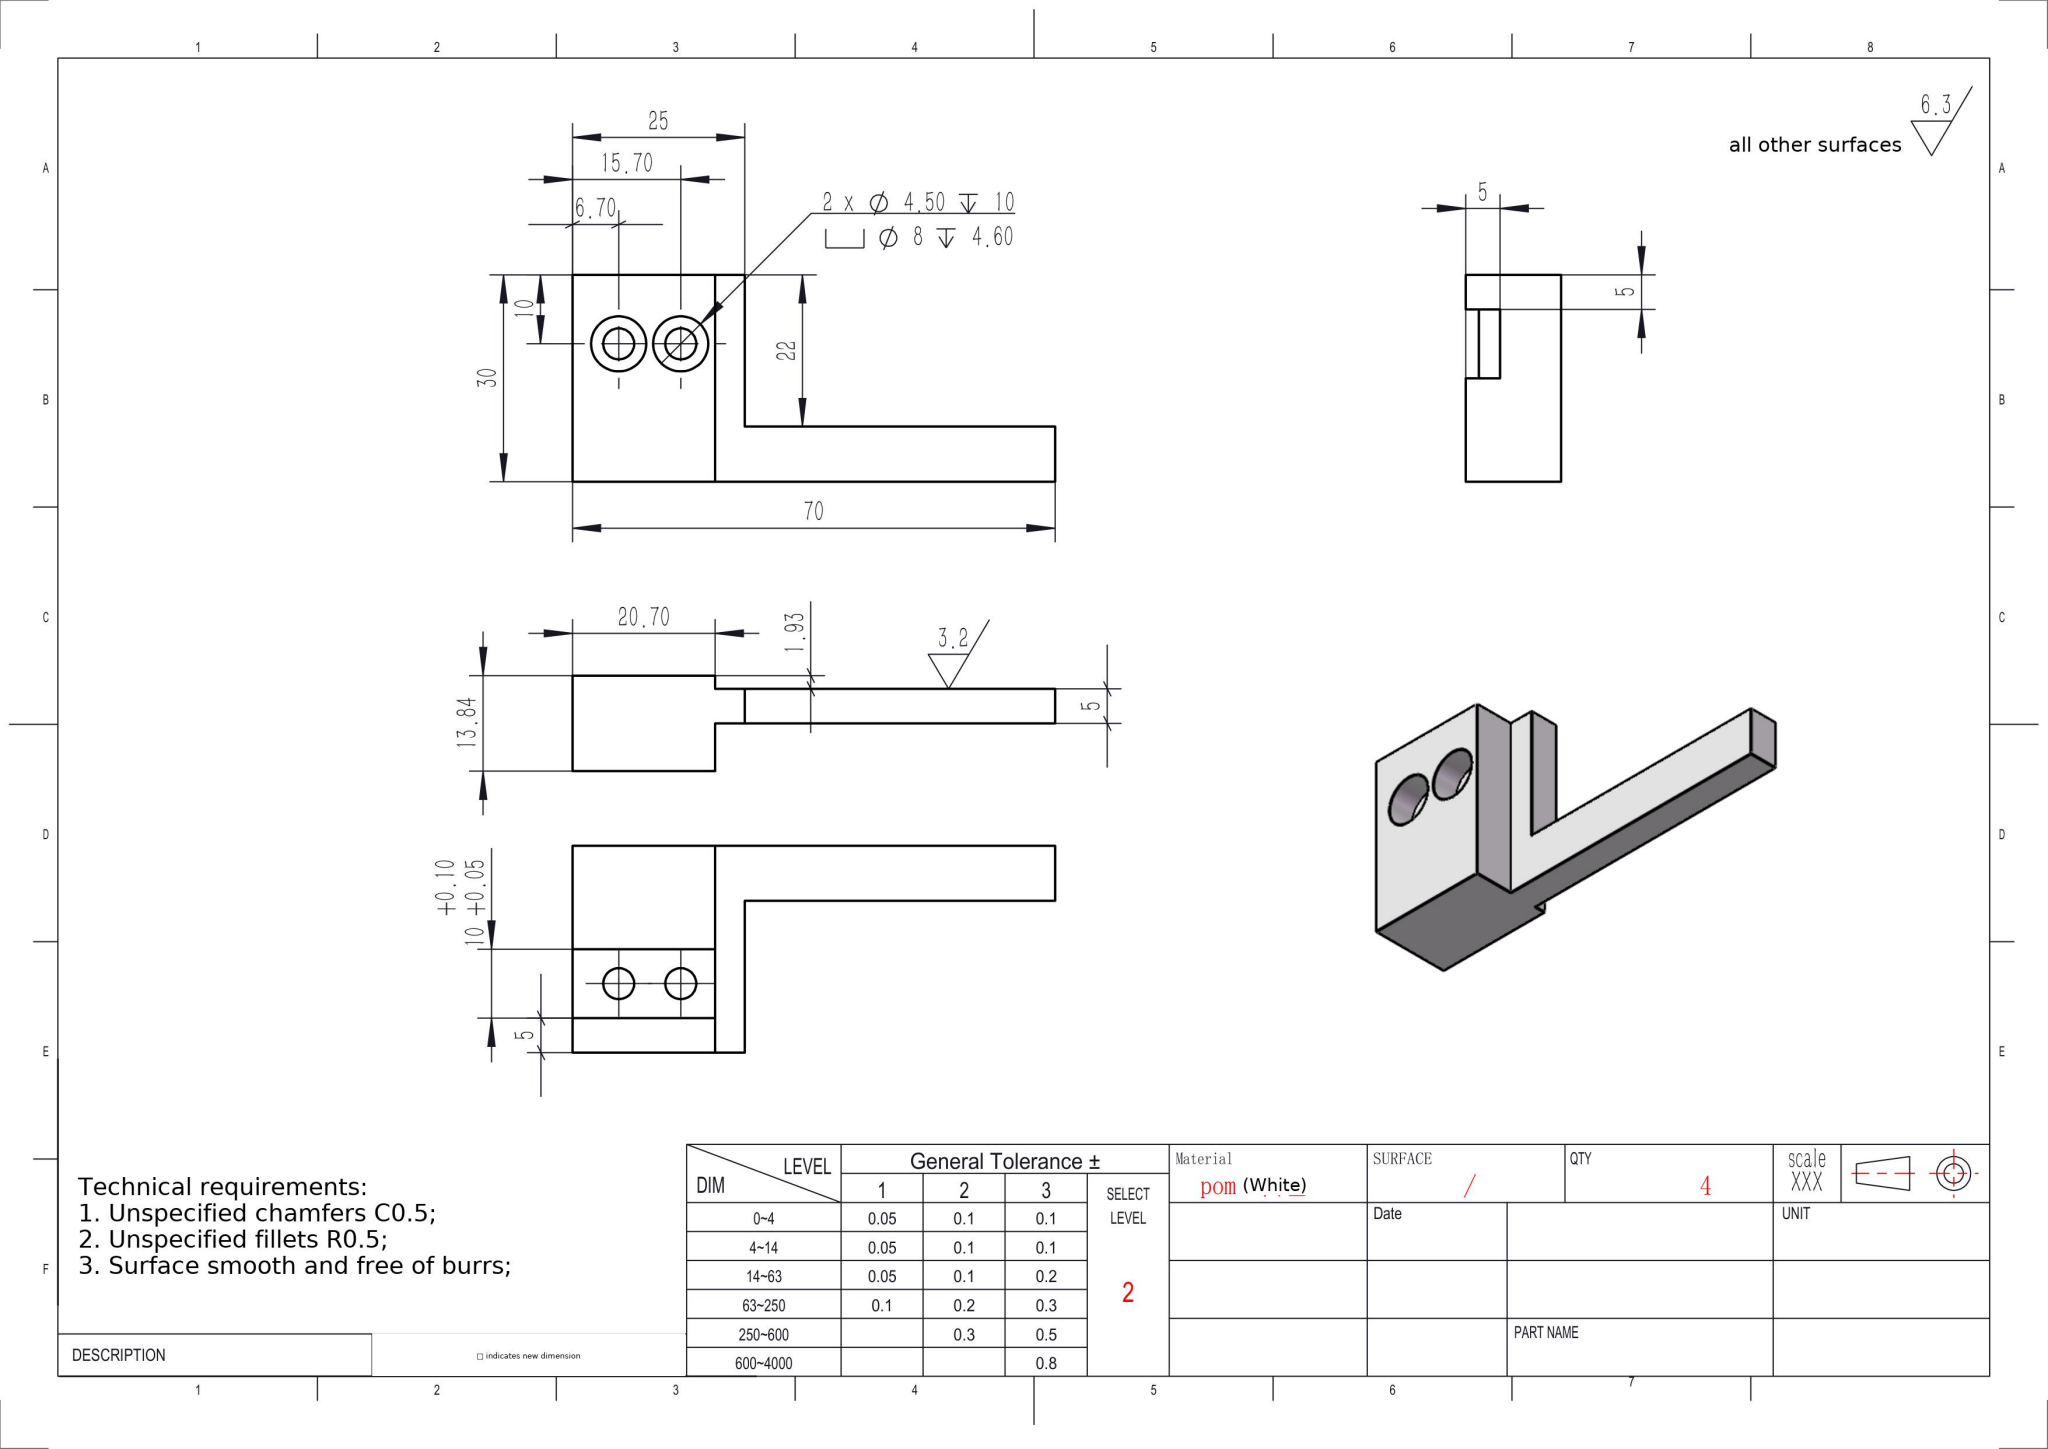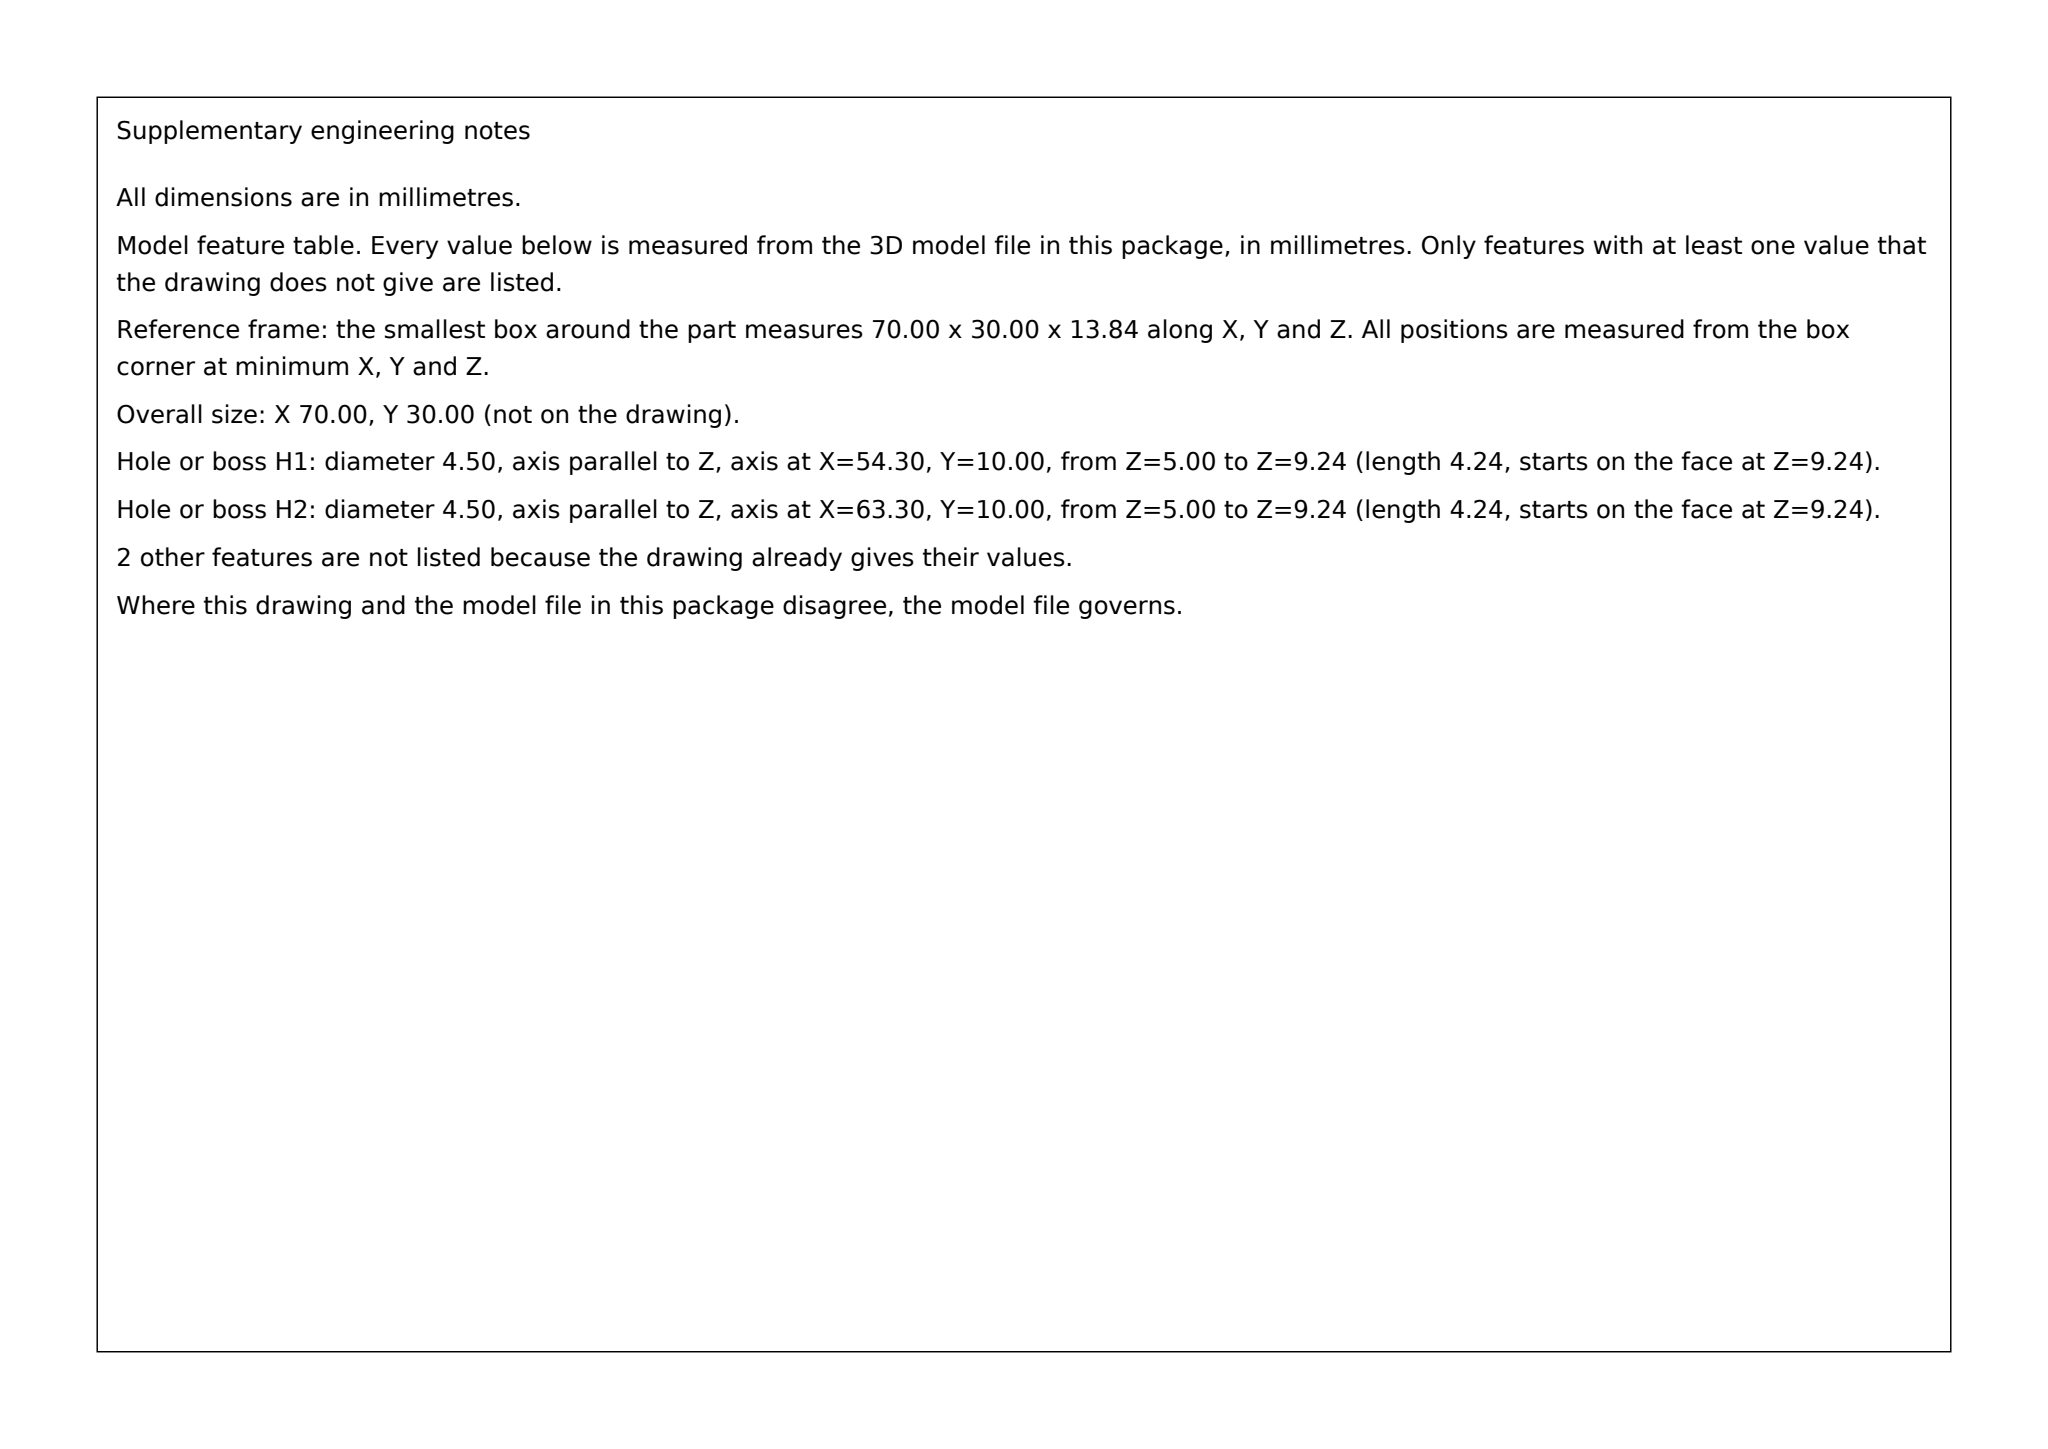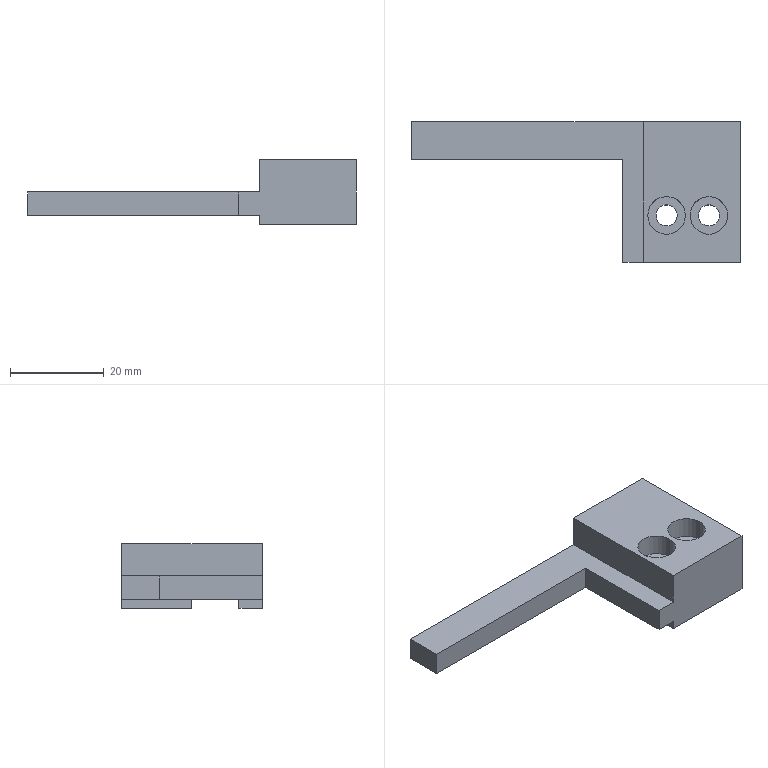Part | SolidWorks | mm | material pom (White) | 1 solid | 28 faces | box 70 x 30 x 13.84 mm | volume 9407 mm3 | plane 20 | cylinder 8 | commonest cylinder face diameters 4.5 x4 8 x4
build123d program:
from build123d import *

# Parameters (mm, degrees)
SKETCH1_W                                         = 50
SKETCH1_H                                         = 30
BOSS_EXTRUDE1_DEPTH                               = 70
SKETCH2_W                                         = 32.32
SKETCH2_H                                         = 10
CUT_EXTRUDE1_DEPTH                                = 20.7
HOLE_SIZE_ACCORDING_TO_HEXAGON_SOCKET_D           = 4.5
HOLE_SIZE_ACCORDING_TO_HEXAGON_SOCKET_DEPTH       = 10
HOLE_SIZE_ACCORDING_TO_HEXAGON_SOCKET_CBORE_D     = 8
HOLE_SIZE_ACCORDING_TO_HEXAGON_SOCKET_CBORE_DEPTH = 4.6
HOLE_SIZE_ACCORDING_TO_HEXAGON_SOCKET_TIP         = 1.352
HOLE_SIZE_ACCORDING_TO_HEXAGON_SO_2_D             = 4.5
HOLE_SIZE_ACCORDING_TO_HEXAGON_SO_2_DEPTH         = 10
HOLE_SIZE_ACCORDING_TO_HEXAGON_SO_2_CBORE_D       = 8
HOLE_SIZE_ACCORDING_TO_HEXAGON_SO_2_CBORE_DEPTH   = 4.6
HOLE_SIZE_ACCORDING_TO_HEXAGON_SO_2_TIP           = 1.352
SKETCH9_W                                         = 20.7
SKETCH9_H                                         = 22.32
CUT_EXTRUDE4_DEPTH                                = 81.156
SKETCH14_W                                        = 49.3
SKETCH14_H                                        = 26.17
CUT_EXTRUDE8_DEPTH                                = 81.156
SKETCH15_W                                        = 45
SKETCH15_H                                        = 22
CUT_EXTRUDE9_DEPTH                                = 88.321
SKETCH16_W                                        = 70
SKETCH16_H                                        = 13.84
CUT_EXTRUDE10_DEPTH                               = 81.156
SKETCH17_W                                        = 49.3
SKETCH17_H                                        = 6.915
CUT_EXTRUDE11_DEPTH                               = 81.156


with BuildPart() as part:
    # Sketch1 → Boss-Extrude1 (new body)
    with BuildSketch(Plane(origin=(0, 0, 0), x_dir=(0, 0, -1), z_dir=(1, 0, 0))):
        Rectangle(SKETCH1_W, SKETCH1_H)
    extrude(amount=BOSS_EXTRUDE1_DEPTH)

    # Sketch2 → Cut-Extrude1 (cut)
    with BuildSketch(Plane(origin=(70, 0, 0), x_dir=(0, 0, -1), z_dir=(1, 0, 0))):
        with Locations((0, -5)):
            Rectangle(SKETCH2_W, SKETCH2_H)
    extrude(amount=-CUT_EXTRUDE1_DEPTH, mode=Mode.SUBTRACT)

    # Hole Size _ according to_ Hexagon Socket
    with Locations(Plane(origin=(0, 0, -25), x_dir=(-1, 0, 0), z_dir=(0, 0, -1))):
        with Locations((-63.3, -5), (-54.3, -5)):
            CounterBoreHole(HOLE_SIZE_ACCORDING_TO_HEXAGON_SOCKET_D / 2, HOLE_SIZE_ACCORDING_TO_HEXAGON_SOCKET_CBORE_D / 2, HOLE_SIZE_ACCORDING_TO_HEXAGON_SOCKET_CBORE_DEPTH, depth=HOLE_SIZE_ACCORDING_TO_HEXAGON_SOCKET_DEPTH)
            with Locations((0, 0, -(HOLE_SIZE_ACCORDING_TO_HEXAGON_SOCKET_DEPTH + HOLE_SIZE_ACCORDING_TO_HEXAGON_SOCKET_TIP / 2))):  # 118° drill point
                Cone(0, HOLE_SIZE_ACCORDING_TO_HEXAGON_SOCKET_D / 2, HOLE_SIZE_ACCORDING_TO_HEXAGON_SOCKET_TIP, mode=Mode.SUBTRACT)

    # Hole Size _ according to_ Hexagon So 2
    with Locations(Plane.XY.offset(25)):
        with Locations((63.3, -5), (54.3, -5)):
            CounterBoreHole(HOLE_SIZE_ACCORDING_TO_HEXAGON_SO_2_D / 2, HOLE_SIZE_ACCORDING_TO_HEXAGON_SO_2_CBORE_D / 2, HOLE_SIZE_ACCORDING_TO_HEXAGON_SO_2_CBORE_DEPTH, depth=HOLE_SIZE_ACCORDING_TO_HEXAGON_SO_2_DEPTH)
            with Locations((0, 0, -(HOLE_SIZE_ACCORDING_TO_HEXAGON_SO_2_DEPTH + HOLE_SIZE_ACCORDING_TO_HEXAGON_SO_2_TIP / 2))):  # 118° drill point
                Cone(0, HOLE_SIZE_ACCORDING_TO_HEXAGON_SO_2_D / 2, HOLE_SIZE_ACCORDING_TO_HEXAGON_SO_2_TIP, mode=Mode.SUBTRACT)

    # Sketch9 → Cut-Extrude4 (cut, through all)
    with BuildSketch(Plane(origin=(0, 15, 0), x_dir=(1, 0, 0), z_dir=(0, 1, 0))):
        with Locations((59.65, 0)):
            Rectangle(SKETCH9_W, SKETCH9_H)
    extrude(amount=-CUT_EXTRUDE4_DEPTH, mode=Mode.SUBTRACT)

    # Sketch14 → Cut-Extrude8 (cut, through all)
    with BuildSketch(Plane(origin=(0, 15, 0), x_dir=(1, 0, 0), z_dir=(0, 1, 0))):
        with Locations((24.65, 0)):
            Rectangle(SKETCH14_W, SKETCH14_H)
    extrude(amount=-CUT_EXTRUDE8_DEPTH, mode=Mode.SUBTRACT)


with BuildPart() as cut_extrude8_piece_1:
    # of the separate pieces the step leaves, piece 1, a body of its own (cut_extrude8_pieces)
    add(part.part.solids().sort_by_distance((0, 15, 25))[0])


with BuildPart() as cut_extrude8_piece_2:
    # of the separate pieces the step leaves, piece 2, a body of its own (cut_extrude8_pieces)
    add(part.part.solids().sort_by_distance((0, 15, -13.085))[0])


with BuildPart() as cut_extrude9_tool:
    # Sketch15 → Cut-Extrude9 (new, through all)
    with BuildSketch(Plane(origin=(0, 0, -25), x_dir=(-1, 0, 0), z_dir=(0, 0, -1))):
        with Locations((-22.5, -4)):
            Rectangle(SKETCH15_W, SKETCH15_H)
    extrude(amount=-CUT_EXTRUDE9_DEPTH)


with BuildPart() as cut_extrude8_piece_1_1:
    add(cut_extrude8_piece_1.part)

    # Cut-Extrude9: cut by cut_extrude9_tool
    add(cut_extrude9_tool.part, mode=Mode.SUBTRACT)

    # Sketch17 → Cut-Extrude11 (cut, through all)
    with BuildSketch(Plane(origin=(0, 15, 0), x_dir=(1, 0, 0), z_dir=(0, 1, 0))):
        with Locations((24.65, -21.543)):
            Rectangle(SKETCH17_W, SKETCH17_H)
    extrude(amount=-CUT_EXTRUDE11_DEPTH, mode=Mode.SUBTRACT)


with BuildPart() as cut_extrude8_piece_2_1:
    add(cut_extrude8_piece_2.part)

    # Cut-Extrude9: cut by cut_extrude9_tool
    add(cut_extrude9_tool.part, mode=Mode.SUBTRACT)

    # Sketch16 → Cut-Extrude10 (cut, through all)
    with BuildSketch(Plane.XZ.offset(15)):
        with Locations((35, -18.08)):
            Rectangle(SKETCH16_W, SKETCH16_H)
    extrude(amount=-CUT_EXTRUDE10_DEPTH, mode=Mode.SUBTRACT)


solid = cut_extrude8_piece_1_1.part
STEP:
#1=CARTESIAN_POINT('',(61.05,-5.,16.16));
#2=VERTEX_POINT('',#1);
#3=CARTESIAN_POINT('',(65.55,-5.,16.16));
#4=VERTEX_POINT('',#3);
#5=CARTESIAN_POINT('',(63.3,-5.,16.16));
#6=DIRECTION('',(0.,0.,1.));
#7=DIRECTION('',(1.,0.,0.));
#8=AXIS2_PLACEMENT_3D('',#5,#6,#7);
#9=CIRCLE('',#8,2.25);
#10=EDGE_CURVE('',#2,#4,#9,.T.);
#11=ORIENTED_EDGE('',*,*,#10,.F.);
#12=CARTESIAN_POINT('',(61.05,-5.,20.4));
#13=VERTEX_POINT('',#12);
#14=CARTESIAN_POINT('',(61.05,-5.,25.));
#15=DIRECTION('',(0.,0.,1.));
#16=VECTOR('',#15,1000.);
#17=LINE('',#14,#16);
#18=EDGE_CURVE('',#2,#13,#17,.T.);
#19=ORIENTED_EDGE('',*,*,#18,.T.);
#20=CARTESIAN_POINT('',(65.55,-5.,20.4));
#21=VERTEX_POINT('',#20);
#22=CARTESIAN_POINT('',(63.3,-5.,20.4));
#23=DIRECTION('',(0.,0.,1.));
#24=DIRECTION('',(1.,0.,0.));
#25=AXIS2_PLACEMENT_3D('',#22,#23,#24);
#26=CIRCLE('',#25,2.25);
#27=EDGE_CURVE('',#13,#21,#26,.T.);
#28=ORIENTED_EDGE('',*,*,#27,.T.);
#29=CARTESIAN_POINT('',(65.55,-5.,25.));
#30=DIRECTION('',(0.,0.,1.));
#31=VECTOR('',#30,1000.);
#32=LINE('',#29,#31);
#33=EDGE_CURVE('',#4,#21,#32,.T.);
#34=ORIENTED_EDGE('',*,*,#33,.F.);
#35=EDGE_LOOP('',(#11,#19,#28,#34));
#36=FACE_OUTER_BOUND('',#35,.T.);
#37=CARTESIAN_POINT('',(63.3,-5.,25.));
#38=DIRECTION('',(0.,0.,1.));
#39=DIRECTION('',(1.,0.,0.));
#40=AXIS2_PLACEMENT_3D('',#37,#38,#39);
#41=CYLINDRICAL_SURFACE('',#40,2.25);
#42=ADVANCED_FACE('',(#36),#41,.F.);
#43=CARTESIAN_POINT('',(52.05,-5.,16.16));
#44=VERTEX_POINT('',#43);
#45=CARTESIAN_POINT('',(56.55,-5.,16.16));
#46=VERTEX_POINT('',#45);
#47=CARTESIAN_POINT('',(54.3,-5.,16.16));
#48=DIRECTION('',(0.,0.,1.));
#49=DIRECTION('',(1.,0.,0.));
#50=AXIS2_PLACEMENT_3D('',#47,#48,#49);
#51=CIRCLE('',#50,2.25);
#52=EDGE_CURVE('',#44,#46,#51,.T.);
#53=ORIENTED_EDGE('',*,*,#52,.F.);
#54=CARTESIAN_POINT('',(52.05,-5.,20.4));
#55=VERTEX_POINT('',#54);
#56=CARTESIAN_POINT('',(52.05,-5.,25.));
#57=DIRECTION('',(0.,0.,1.));
#58=VECTOR('',#57,1000.);
#59=LINE('',#56,#58);
#60=EDGE_CURVE('',#44,#55,#59,.T.);
#61=ORIENTED_EDGE('',*,*,#60,.T.);
#62=CARTESIAN_POINT('',(56.55,-5.,20.4));
#63=VERTEX_POINT('',#62);
#64=CARTESIAN_POINT('',(54.3,-5.,20.4));
#65=DIRECTION('',(0.,0.,1.));
#66=DIRECTION('',(1.,0.,0.));
#67=AXIS2_PLACEMENT_3D('',#64,#65,#66);
#68=CIRCLE('',#67,2.25);
#69=EDGE_CURVE('',#55,#63,#68,.T.);
#70=ORIENTED_EDGE('',*,*,#69,.T.);
#71=CARTESIAN_POINT('',(56.55,-5.,25.));
#72=DIRECTION('',(0.,0.,1.));
#73=VECTOR('',#72,1000.);
#74=LINE('',#71,#73);
#75=EDGE_CURVE('',#46,#63,#74,.T.);
#76=ORIENTED_EDGE('',*,*,#75,.F.);
#77=EDGE_LOOP('',(#53,#61,#70,#76));
#78=FACE_OUTER_BOUND('',#77,.T.);
#79=CARTESIAN_POINT('',(54.3,-5.,25.));
#80=DIRECTION('',(0.,0.,1.));
#81=DIRECTION('',(1.,0.,0.));
#82=AXIS2_PLACEMENT_3D('',#79,#80,#81);
#83=CYLINDRICAL_SURFACE('',#82,2.25);
#84=ADVANCED_FACE('',(#78),#83,.F.);
#85=CARTESIAN_POINT('',(59.3,-5.,20.4));
#86=VERTEX_POINT('',#85);
#87=CARTESIAN_POINT('',(67.3,-5.,20.4));
#88=VERTEX_POINT('',#87);
#89=CARTESIAN_POINT('',(63.3,-5.,20.4));
#90=DIRECTION('',(0.,0.,1.));
#91=DIRECTION('',(1.,0.,0.));
#92=AXIS2_PLACEMENT_3D('',#89,#90,#91);
#93=CIRCLE('',#92,4.);
#94=EDGE_CURVE('',#86,#88,#93,.T.);
#95=ORIENTED_EDGE('',*,*,#94,.F.);
#96=CARTESIAN_POINT('',(59.3,-5.,25.));
#97=VERTEX_POINT('',#96);
#98=CARTESIAN_POINT('',(59.3,-5.,25.));
#99=DIRECTION('',(0.,0.,1.));
#100=VECTOR('',#99,1000.);
#101=LINE('',#98,#100);
#102=EDGE_CURVE('',#86,#97,#101,.T.);
#103=ORIENTED_EDGE('',*,*,#102,.T.);
#104=CARTESIAN_POINT('',(67.3,-5.,25.));
#105=VERTEX_POINT('',#104);
#106=CARTESIAN_POINT('',(63.3,-5.,25.));
#107=DIRECTION('',(0.,0.,1.));
#108=DIRECTION('',(1.,0.,0.));
#109=AXIS2_PLACEMENT_3D('',#106,#107,#108);
#110=CIRCLE('',#109,4.);
#111=EDGE_CURVE('',#97,#105,#110,.T.);
#112=ORIENTED_EDGE('',*,*,#111,.T.);
#113=CARTESIAN_POINT('',(67.3,-5.,25.));
#114=DIRECTION('',(0.,0.,1.));
#115=VECTOR('',#114,1000.);
#116=LINE('',#113,#115);
#117=EDGE_CURVE('',#88,#105,#116,.T.);
#118=ORIENTED_EDGE('',*,*,#117,.F.);
#119=EDGE_LOOP('',(#95,#103,#112,#118));
#120=FACE_OUTER_BOUND('',#119,.T.);
#121=CARTESIAN_POINT('',(63.3,-5.,25.));
#122=DIRECTION('',(0.,0.,1.));
#123=DIRECTION('',(1.,0.,0.));
#124=AXIS2_PLACEMENT_3D('',#121,#122,#123);
#125=CYLINDRICAL_SURFACE('',#124,4.);
#126=ADVANCED_FACE('',(#120),#125,.F.);
#127=CARTESIAN_POINT('',(50.3,-5.,20.4));
#128=VERTEX_POINT('',#127);
#129=CARTESIAN_POINT('',(58.3,-5.,20.4));
#130=VERTEX_POINT('',#129);
#131=CARTESIAN_POINT('',(54.3,-5.,20.4));
#132=DIRECTION('',(0.,0.,1.));
#133=DIRECTION('',(1.,0.,0.));
#134=AXIS2_PLACEMENT_3D('',#131,#132,#133);
#135=CIRCLE('',#134,4.);
#136=EDGE_CURVE('',#128,#130,#135,.T.);
#137=ORIENTED_EDGE('',*,*,#136,.F.);
#138=CARTESIAN_POINT('',(50.3,-5.,25.));
#139=VERTEX_POINT('',#138);
#140=CARTESIAN_POINT('',(50.3,-5.,25.));
#141=DIRECTION('',(0.,0.,1.));
#142=VECTOR('',#141,1000.);
#143=LINE('',#140,#142);
#144=EDGE_CURVE('',#128,#139,#143,.T.);
#145=ORIENTED_EDGE('',*,*,#144,.T.);
#146=CARTESIAN_POINT('',(58.3,-5.,25.));
#147=VERTEX_POINT('',#146);
#148=CARTESIAN_POINT('',(54.3,-5.,25.));
#149=DIRECTION('',(0.,0.,1.));
#150=DIRECTION('',(1.,0.,0.));
#151=AXIS2_PLACEMENT_3D('',#148,#149,#150);
#152=CIRCLE('',#151,4.);
#153=EDGE_CURVE('',#139,#147,#152,.T.);
#154=ORIENTED_EDGE('',*,*,#153,.T.);
#155=CARTESIAN_POINT('',(58.3,-5.,25.));
#156=DIRECTION('',(0.,0.,1.));
#157=VECTOR('',#156,1000.);
#158=LINE('',#155,#157);
#159=EDGE_CURVE('',#130,#147,#158,.T.);
#160=ORIENTED_EDGE('',*,*,#159,.F.);
#161=EDGE_LOOP('',(#137,#145,#154,#160));
#162=FACE_OUTER_BOUND('',#161,.T.);
#163=CARTESIAN_POINT('',(54.3,-5.,25.));
#164=DIRECTION('',(0.,0.,1.));
#165=DIRECTION('',(1.,0.,0.));
#166=AXIS2_PLACEMENT_3D('',#163,#164,#165);
#167=CYLINDRICAL_SURFACE('',#166,4.);
#168=ADVANCED_FACE('',(#162),#167,.F.);
#169=CARTESIAN_POINT('',(54.3,-5.,20.4));
#170=DIRECTION('',(0.,0.,1.));
#171=DIRECTION('',(1.,0.,0.));
#172=AXIS2_PLACEMENT_3D('',#169,#170,#171);
#173=CIRCLE('',#172,2.25);
#174=EDGE_CURVE('',#63,#55,#173,.T.);
#175=ORIENTED_EDGE('',*,*,#174,.F.);
#176=ORIENTED_EDGE('',*,*,#69,.F.);
#177=EDGE_LOOP('',(#175,#176));
#178=FACE_BOUND('',#177,.T.);
#179=CARTESIAN_POINT('',(54.3,-5.,20.4));
#180=DIRECTION('',(0.,0.,1.));
#181=DIRECTION('',(1.,0.,0.));
#182=AXIS2_PLACEMENT_3D('',#179,#180,#181);
#183=CIRCLE('',#182,4.);
#184=EDGE_CURVE('',#130,#128,#183,.T.);
#185=ORIENTED_EDGE('',*,*,#184,.T.);
#186=ORIENTED_EDGE('',*,*,#136,.T.);
#187=EDGE_LOOP('',(#185,#186));
#188=FACE_OUTER_BOUND('',#187,.T.);
#189=CARTESIAN_POINT('',(56.55,-5.,20.4));
#190=DIRECTION('',(0.,0.,-1.));
#191=DIRECTION('',(-1.,0.,0.));
#192=AXIS2_PLACEMENT_3D('',#189,#190,#191);
#193=PLANE('',#192);
#194=ADVANCED_FACE('',(#178,#188),#193,.F.);
#195=CARTESIAN_POINT('',(63.3,-5.,20.4));
#196=DIRECTION('',(0.,0.,1.));
#197=DIRECTION('',(1.,0.,0.));
#198=AXIS2_PLACEMENT_3D('',#195,#196,#197);
#199=CIRCLE('',#198,2.25);
#200=EDGE_CURVE('',#21,#13,#199,.T.);
#201=ORIENTED_EDGE('',*,*,#200,.F.);
#202=ORIENTED_EDGE('',*,*,#27,.F.);
#203=EDGE_LOOP('',(#201,#202));
#204=FACE_BOUND('',#203,.T.);
#205=CARTESIAN_POINT('',(63.3,-5.,20.4));
#206=DIRECTION('',(0.,0.,1.));
#207=DIRECTION('',(1.,0.,0.));
#208=AXIS2_PLACEMENT_3D('',#205,#206,#207);
#209=CIRCLE('',#208,4.);
#210=EDGE_CURVE('',#88,#86,#209,.T.);
#211=ORIENTED_EDGE('',*,*,#210,.T.);
#212=ORIENTED_EDGE('',*,*,#94,.T.);
#213=EDGE_LOOP('',(#211,#212));
#214=FACE_OUTER_BOUND('',#213,.T.);
#215=CARTESIAN_POINT('',(65.55,-5.,20.4));
#216=DIRECTION('',(0.,0.,-1.));
#217=DIRECTION('',(-1.,0.,0.));
#218=AXIS2_PLACEMENT_3D('',#215,#216,#217);
#219=PLANE('',#218);
#220=ADVANCED_FACE('',(#204,#214),#219,.F.);
#221=ORIENTED_EDGE('',*,*,#144,.F.);
#222=ORIENTED_EDGE('',*,*,#184,.F.);
#223=ORIENTED_EDGE('',*,*,#159,.T.);
#224=CARTESIAN_POINT('',(54.3,-5.,25.));
#225=DIRECTION('',(0.,0.,1.));
#226=DIRECTION('',(1.,0.,0.));
#227=AXIS2_PLACEMENT_3D('',#224,#225,#226);
#228=CIRCLE('',#227,4.);
#229=EDGE_CURVE('',#147,#139,#228,.T.);
#230=ORIENTED_EDGE('',*,*,#229,.T.);
#231=EDGE_LOOP('',(#221,#222,#223,#230));
#232=FACE_OUTER_BOUND('',#231,.T.);
#233=CARTESIAN_POINT('',(54.3,-5.,25.));
#234=DIRECTION('',(0.,0.,1.));
#235=DIRECTION('',(1.,0.,0.));
#236=AXIS2_PLACEMENT_3D('',#233,#234,#235);
#237=CYLINDRICAL_SURFACE('',#236,4.);
#238=ADVANCED_FACE('',(#232),#237,.F.);
#239=ORIENTED_EDGE('',*,*,#102,.F.);
#240=ORIENTED_EDGE('',*,*,#210,.F.);
#241=ORIENTED_EDGE('',*,*,#117,.T.);
#242=CARTESIAN_POINT('',(63.3,-5.,25.));
#243=DIRECTION('',(0.,0.,1.));
#244=DIRECTION('',(1.,0.,0.));
#245=AXIS2_PLACEMENT_3D('',#242,#243,#244);
#246=CIRCLE('',#245,4.);
#247=EDGE_CURVE('',#105,#97,#246,.T.);
#248=ORIENTED_EDGE('',*,*,#247,.T.);
#249=EDGE_LOOP('',(#239,#240,#241,#248));
#250=FACE_OUTER_BOUND('',#249,.T.);
#251=CARTESIAN_POINT('',(63.3,-5.,25.));
#252=DIRECTION('',(0.,0.,1.));
#253=DIRECTION('',(1.,0.,0.));
#254=AXIS2_PLACEMENT_3D('',#251,#252,#253);
#255=CYLINDRICAL_SURFACE('',#254,4.);
#256=ADVANCED_FACE('',(#250),#255,.F.);
#257=ORIENTED_EDGE('',*,*,#60,.F.);
#258=CARTESIAN_POINT('',(54.3,-5.,16.16));
#259=DIRECTION('',(0.,0.,1.));
#260=DIRECTION('',(1.,0.,0.));
#261=AXIS2_PLACEMENT_3D('',#258,#259,#260);
#262=CIRCLE('',#261,2.25);
#263=EDGE_CURVE('',#46,#44,#262,.T.);
#264=ORIENTED_EDGE('',*,*,#263,.F.);
#265=ORIENTED_EDGE('',*,*,#75,.T.);
#266=ORIENTED_EDGE('',*,*,#174,.T.);
#267=EDGE_LOOP('',(#257,#264,#265,#266));
#268=FACE_OUTER_BOUND('',#267,.T.);
#269=CARTESIAN_POINT('',(54.3,-5.,25.));
#270=DIRECTION('',(0.,0.,1.));
#271=DIRECTION('',(1.,0.,0.));
#272=AXIS2_PLACEMENT_3D('',#269,#270,#271);
#273=CYLINDRICAL_SURFACE('',#272,2.25);
#274=ADVANCED_FACE('',(#268),#273,.F.);
#275=ORIENTED_EDGE('',*,*,#18,.F.);
#276=CARTESIAN_POINT('',(63.3,-5.,16.16));
#277=DIRECTION('',(0.,0.,1.));
#278=DIRECTION('',(1.,0.,0.));
#279=AXIS2_PLACEMENT_3D('',#276,#277,#278);
#280=CIRCLE('',#279,2.25);
#281=EDGE_CURVE('',#4,#2,#280,.T.);
#282=ORIENTED_EDGE('',*,*,#281,.F.);
#283=ORIENTED_EDGE('',*,*,#33,.T.);
#284=ORIENTED_EDGE('',*,*,#200,.T.);
#285=EDGE_LOOP('',(#275,#282,#283,#284));
#286=FACE_OUTER_BOUND('',#285,.T.);
#287=CARTESIAN_POINT('',(63.3,-5.,25.));
#288=DIRECTION('',(0.,0.,1.));
#289=DIRECTION('',(1.,0.,0.));
#290=AXIS2_PLACEMENT_3D('',#287,#288,#289);
#291=CYLINDRICAL_SURFACE('',#290,2.25);
#292=ADVANCED_FACE('',(#286),#291,.F.);
#293=ORIENTED_EDGE('',*,*,#247,.F.);
#294=ORIENTED_EDGE('',*,*,#111,.F.);
#295=EDGE_LOOP('',(#293,#294));
#296=FACE_BOUND('',#295,.T.);
#297=ORIENTED_EDGE('',*,*,#229,.F.);
#298=ORIENTED_EDGE('',*,*,#153,.F.);
#299=EDGE_LOOP('',(#297,#298));
#300=FACE_BOUND('',#299,.T.);
#301=CARTESIAN_POINT('',(70.,15.,25.));
#302=VERTEX_POINT('',#301);
#303=CARTESIAN_POINT('',(49.3,15.,25.));
#304=VERTEX_POINT('',#303);
#305=CARTESIAN_POINT('',(70.,15.,25.));
#306=DIRECTION('',(-1.,0.,0.));
#307=VECTOR('',#306,1000.);
#308=LINE('',#305,#307);
#309=EDGE_CURVE('',#302,#304,#308,.T.);
#310=ORIENTED_EDGE('',*,*,#309,.T.);
#311=CARTESIAN_POINT('',(49.3,-15.,25.));
#312=VERTEX_POINT('',#311);
#313=CARTESIAN_POINT('',(49.3,-15.,25.));
#314=DIRECTION('',(0.,1.,0.));
#315=VECTOR('',#314,1000.);
#316=LINE('',#313,#315);
#317=EDGE_CURVE('',#312,#304,#316,.T.);
#318=ORIENTED_EDGE('',*,*,#317,.F.);
#319=CARTESIAN_POINT('',(70.,-15.,25.));
#320=VERTEX_POINT('',#319);
#321=CARTESIAN_POINT('',(70.,-15.,25.));
#322=DIRECTION('',(-1.,0.,0.));
#323=VECTOR('',#322,1000.);
#324=LINE('',#321,#323);
#325=EDGE_CURVE('',#320,#312,#324,.T.);
#326=ORIENTED_EDGE('',*,*,#325,.F.);
#327=CARTESIAN_POINT('',(70.,15.,25.));
#328=DIRECTION('',(0.,-1.,-0.));
#329=VECTOR('',#328,1000.);
#330=LINE('',#327,#329);
#331=EDGE_CURVE('',#302,#320,#330,.T.);
#332=ORIENTED_EDGE('',*,*,#331,.F.);
#333=EDGE_LOOP('',(#310,#318,#326,#332));
#334=FACE_OUTER_BOUND('',#333,.T.);
#335=CARTESIAN_POINT('',(70.,15.,25.));
#336=DIRECTION('',(0.,0.,-1.));
#337=DIRECTION('',(0.,1.,0.));
#338=AXIS2_PLACEMENT_3D('',#335,#336,#337);
#339=PLANE('',#338);
#340=ADVANCED_FACE('',(#296,#300,#334),#339,.F.);
#341=ORIENTED_EDGE('',*,*,#281,.T.);
#342=ORIENTED_EDGE('',*,*,#10,.T.);
#343=EDGE_LOOP('',(#341,#342));
#344=FACE_BOUND('',#343,.T.);
#345=ORIENTED_EDGE('',*,*,#263,.T.);
#346=ORIENTED_EDGE('',*,*,#52,.T.);
#347=EDGE_LOOP('',(#345,#346));
#348=FACE_BOUND('',#347,.T.);
#349=CARTESIAN_POINT('',(70.,-0.,16.16));
#350=VERTEX_POINT('',#349);
#351=CARTESIAN_POINT('',(70.,-10.,16.16));
#352=VERTEX_POINT('',#351);
#353=CARTESIAN_POINT('',(70.,-0.,16.16));
#354=DIRECTION('',(0.,-1.,0.));
#355=VECTOR('',#354,1000.);
#356=LINE('',#353,#355);
#357=EDGE_CURVE('',#350,#352,#356,.T.);
#358=ORIENTED_EDGE('',*,*,#357,.T.);
#359=CARTESIAN_POINT('',(49.3,-10.,16.16));
#360=VERTEX_POINT('',#359);
#361=CARTESIAN_POINT('',(49.3,-10.,16.16));
#362=DIRECTION('',(1.,0.,0.));
#363=VECTOR('',#362,1000.);
#364=LINE('',#361,#363);
#365=EDGE_CURVE('',#360,#352,#364,.T.);
#366=ORIENTED_EDGE('',*,*,#365,.F.);
#367=CARTESIAN_POINT('',(49.3,-0.,16.16));
#368=VERTEX_POINT('',#367);
#369=CARTESIAN_POINT('',(49.3,-0.,16.16));
#370=DIRECTION('',(0.,-1.,0.));
#371=VECTOR('',#370,1000.);
#372=LINE('',#369,#371);
#373=EDGE_CURVE('',#368,#360,#372,.T.);
#374=ORIENTED_EDGE('',*,*,#373,.F.);
#375=CARTESIAN_POINT('',(49.3,-0.,16.16));
#376=DIRECTION('',(1.,0.,0.));
#377=VECTOR('',#376,1000.);
#378=LINE('',#375,#377);
#379=EDGE_CURVE('',#368,#350,#378,.T.);
#380=ORIENTED_EDGE('',*,*,#379,.T.);
#381=EDGE_LOOP('',(#358,#366,#374,#380));
#382=FACE_OUTER_BOUND('',#381,.T.);
#383=CARTESIAN_POINT('',(49.3,-0.,16.16));
#384=DIRECTION('',(0.,0.,1.));
#385=DIRECTION('',(1.,0.,0.));
#386=AXIS2_PLACEMENT_3D('',#383,#384,#385);
#387=PLANE('',#386);
#388=ADVANCED_FACE('',(#344,#348,#382),#387,.F.);
#389=CARTESIAN_POINT('',(70.,-0.,11.16));
#390=VERTEX_POINT('',#389);
#391=CARTESIAN_POINT('',(70.,15.,11.16));
#392=VERTEX_POINT('',#391);
#393=CARTESIAN_POINT('',(70.,-15.,11.16));
#394=DIRECTION('',(0.,1.,0.));
#395=VECTOR('',#394,1000.);
#396=LINE('',#393,#395);
#397=EDGE_CURVE('',#390,#392,#396,.T.);
#398=ORIENTED_EDGE('',*,*,#397,.T.);
#399=CARTESIAN_POINT('',(70.,15.,25.));
#400=DIRECTION('',(0.,0.,1.));
#401=VECTOR('',#400,1000.);
#402=LINE('',#399,#401);
#403=EDGE_CURVE('',#392,#302,#402,.T.);
#404=ORIENTED_EDGE('',*,*,#403,.T.);
#405=ORIENTED_EDGE('',*,*,#331,.T.);
#406=CARTESIAN_POINT('',(70.,-15.,11.16));
#407=VERTEX_POINT('',#406);
#408=CARTESIAN_POINT('',(70.,-15.,25.));
#409=DIRECTION('',(0.,0.,-1.));
#410=VECTOR('',#409,1000.);
#411=LINE('',#408,#410);
#412=EDGE_CURVE('',#320,#407,#411,.T.);
#413=ORIENTED_EDGE('',*,*,#412,.T.);
#414=CARTESIAN_POINT('',(70.,-10.,11.16));
#415=VERTEX_POINT('',#414);
#416=CARTESIAN_POINT('',(70.,-15.,11.16));
#417=DIRECTION('',(0.,1.,0.));
#418=VECTOR('',#417,1000.);
#419=LINE('',#416,#418);
#420=EDGE_CURVE('',#407,#415,#419,.T.);
#421=ORIENTED_EDGE('',*,*,#420,.T.);
#422=CARTESIAN_POINT('',(70.,-10.,16.16));
#423=DIRECTION('',(0.,0.,-1.));
#424=VECTOR('',#423,1000.);
#425=LINE('',#422,#424);
#426=EDGE_CURVE('',#352,#415,#425,.T.);
#427=ORIENTED_EDGE('',*,*,#426,.F.);
#428=ORIENTED_EDGE('',*,*,#357,.F.);
#429=CARTESIAN_POINT('',(70.,-0.,16.16));
#430=DIRECTION('',(0.,-0.,1.));
#431=VECTOR('',#430,1000.);
#432=LINE('',#429,#431);
#433=EDGE_CURVE('',#390,#350,#432,.T.);
#434=ORIENTED_EDGE('',*,*,#433,.F.);
#435=EDGE_LOOP('',(#398,#404,#405,#413,#421,#427,#428,#434));
#436=FACE_OUTER_BOUND('',#435,.T.);
#437=CARTESIAN_POINT('',(70.,0.,0.));
#438=DIRECTION('',(1.,0.,0.));
#439=DIRECTION('',(0.,0.,-1.));
#440=AXIS2_PLACEMENT_3D('',#437,#438,#439);
#441=PLANE('',#440);
#442=ADVANCED_FACE('',(#436),#441,.T.);
#443=CARTESIAN_POINT('',(49.3,-10.,13.085));
#444=VERTEX_POINT('',#443);
#445=CARTESIAN_POINT('',(49.3,-0.,13.085));
#446=VERTEX_POINT('',#445);
#447=CARTESIAN_POINT('',(49.3,-15.,13.085));
#448=DIRECTION('',(0.,1.,0.));
#449=VECTOR('',#448,1000.);
#450=LINE('',#447,#449);
#451=EDGE_CURVE('',#444,#446,#450,.T.);
#452=ORIENTED_EDGE('',*,*,#451,.T.);
#453=CARTESIAN_POINT('',(49.3,-0.,16.16));
#454=DIRECTION('',(0.,-0.,1.));
#455=VECTOR('',#454,1000.);
#456=LINE('',#453,#455);
#457=EDGE_CURVE('',#446,#368,#456,.T.);
#458=ORIENTED_EDGE('',*,*,#457,.T.);
#459=ORIENTED_EDGE('',*,*,#373,.T.);
#460=CARTESIAN_POINT('',(49.3,-10.,16.16));
#461=DIRECTION('',(0.,0.,-1.));
#462=VECTOR('',#461,1000.);
#463=LINE('',#460,#462);
#464=EDGE_CURVE('',#360,#444,#463,.T.);
#465=ORIENTED_EDGE('',*,*,#464,.T.);
#466=EDGE_LOOP('',(#452,#458,#459,#465));
#467=FACE_OUTER_BOUND('',#466,.T.);
#468=CARTESIAN_POINT('',(49.3,0.,0.));
#469=DIRECTION('',(1.,0.,0.));
#470=DIRECTION('',(0.,0.,-1.));
#471=AXIS2_PLACEMENT_3D('',#468,#469,#470);
#472=PLANE('',#471);
#473=ADVANCED_FACE('',(#467),#472,.T.);
#474=CARTESIAN_POINT('',(0.,7.,18.085));
#475=VERTEX_POINT('',#474);
#476=CARTESIAN_POINT('',(0.,7.,13.085));
#477=VERTEX_POINT('',#476);
#478=CARTESIAN_POINT('',(0.,7.,25.));
#479=DIRECTION('',(0.,0.,-1.));
#480=VECTOR('',#479,1000.);
#481=LINE('',#478,#480);
#482=EDGE_CURVE('',#475,#477,#481,.T.);
#483=ORIENTED_EDGE('',*,*,#482,.F.);
#484=CARTESIAN_POINT('',(0.,15.,18.085));
#485=VERTEX_POINT('',#484);
#486=CARTESIAN_POINT('',(0.,-15.,18.085));
#487=DIRECTION('',(0.,1.,0.));
#488=VECTOR('',#487,1000.);
#489=LINE('',#486,#488);
#490=EDGE_CURVE('',#475,#485,#489,.T.);
#491=ORIENTED_EDGE('',*,*,#490,.T.);
#492=CARTESIAN_POINT('',(0.,15.,13.085));
#493=VERTEX_POINT('',#492);
#494=CARTESIAN_POINT('',(0.,15.,25.));
#495=DIRECTION('',(0.,0.,1.));
#496=VECTOR('',#495,1000.);
#497=LINE('',#494,#496);
#498=EDGE_CURVE('',#493,#485,#497,.T.);
#499=ORIENTED_EDGE('',*,*,#498,.F.);
#500=CARTESIAN_POINT('',(0.,-15.,13.085));
#501=DIRECTION('',(0.,1.,0.));
#502=VECTOR('',#501,1000.);
#503=LINE('',#500,#502);
#504=EDGE_CURVE('',#477,#493,#503,.T.);
#505=ORIENTED_EDGE('',*,*,#504,.F.);
#506=EDGE_LOOP('',(#483,#491,#499,#505));
#507=FACE_OUTER_BOUND('',#506,.T.);
#508=CARTESIAN_POINT('',(0.,0.,0.));
#509=DIRECTION('',(1.,0.,0.));
#510=DIRECTION('',(0.,0.,-1.));
#511=AXIS2_PLACEMENT_3D('',#508,#509,#510);
#512=PLANE('',#511);
#513=ADVANCED_FACE('',(#507),#512,.F.);
#514=ORIENTED_EDGE('',*,*,#420,.F.);
#515=CARTESIAN_POINT('',(49.3,-15.,11.16));
#516=VERTEX_POINT('',#515);
#517=CARTESIAN_POINT('',(70.,-15.,11.16));
#518=DIRECTION('',(1.,0.,-0.));
#519=VECTOR('',#518,1000.);
#520=LINE('',#517,#519);
#521=EDGE_CURVE('',#516,#407,#520,.T.);
#522=ORIENTED_EDGE('',*,*,#521,.F.);
#523=CARTESIAN_POINT('',(49.3,-10.,11.16));
#524=VERTEX_POINT('',#523);
#525=CARTESIAN_POINT('',(49.3,-15.,11.16));
#526=DIRECTION('',(0.,1.,0.));
#527=VECTOR('',#526,1000.);
#528=LINE('',#525,#527);
#529=EDGE_CURVE('',#516,#524,#528,.T.);
#530=ORIENTED_EDGE('',*,*,#529,.T.);
#531=CARTESIAN_POINT('',(49.3,-10.,11.16));
#532=DIRECTION('',(-1.,0.,0.));
#533=VECTOR('',#532,1000.);
#534=LINE('',#531,#533);
#535=EDGE_CURVE('',#415,#524,#534,.T.);
#536=ORIENTED_EDGE('',*,*,#535,.F.);
#537=EDGE_LOOP('',(#514,#522,#530,#536));
#538=FACE_OUTER_BOUND('',#537,.T.);
#539=CARTESIAN_POINT('',(70.,-15.,11.16));
#540=DIRECTION('',(0.,0.,1.));
#541=DIRECTION('',(1.,0.,-0.));
#542=AXIS2_PLACEMENT_3D('',#539,#540,#541);
#543=PLANE('',#542);
#544=ADVANCED_FACE('',(#538),#543,.F.);
#545=CARTESIAN_POINT('',(49.3,-15.,18.085));
#546=VERTEX_POINT('',#545);
#547=CARTESIAN_POINT('',(49.3,-15.,25.));
#548=DIRECTION('',(0.,0.,-1.));
#549=VECTOR('',#548,1000.);
#550=LINE('',#547,#549);
#551=EDGE_CURVE('',#312,#546,#550,.T.);
#552=ORIENTED_EDGE('',*,*,#551,.T.);
#553=CARTESIAN_POINT('',(45.,-15.,18.085));
#554=VERTEX_POINT('',#553);
#555=CARTESIAN_POINT('',(0.,-15.,18.085));
#556=DIRECTION('',(-1.,0.,0.));
#557=VECTOR('',#556,1000.);
#558=LINE('',#555,#557);
#559=EDGE_CURVE('',#546,#554,#558,.T.);
#560=ORIENTED_EDGE('',*,*,#559,.T.);
#561=CARTESIAN_POINT('',(45.,-15.,13.085));
#562=VERTEX_POINT('',#561);
#563=CARTESIAN_POINT('',(45.,-15.,25.));
#564=DIRECTION('',(0.,0.,-1.));
#565=VECTOR('',#564,1000.);
#566=LINE('',#563,#565);
#567=EDGE_CURVE('',#554,#562,#566,.T.);
#568=ORIENTED_EDGE('',*,*,#567,.T.);
#569=CARTESIAN_POINT('',(49.3,-15.,13.085));
#570=VERTEX_POINT('',#569);
#571=CARTESIAN_POINT('',(0.,-15.,13.085));
#572=DIRECTION('',(1.,0.,0.));
#573=VECTOR('',#572,1000.);
#574=LINE('',#571,#573);
#575=EDGE_CURVE('',#562,#570,#574,.T.);
#576=ORIENTED_EDGE('',*,*,#575,.T.);
#577=CARTESIAN_POINT('',(49.3,-15.,-13.085));
#578=DIRECTION('',(0.,0.,-1.));
#579=VECTOR('',#578,1000.);
#580=LINE('',#577,#579);
#581=EDGE_CURVE('',#570,#516,#580,.T.);
#582=ORIENTED_EDGE('',*,*,#581,.T.);
#583=ORIENTED_EDGE('',*,*,#521,.T.);
#584=ORIENTED_EDGE('',*,*,#412,.F.);
#585=ORIENTED_EDGE('',*,*,#325,.T.);
#586=EDGE_LOOP('',(#552,#560,#568,#576,#582,#583,#584,#585));
#587=FACE_OUTER_BOUND('',#586,.T.);
#588=CARTESIAN_POINT('',(70.,-15.,25.));
#589=DIRECTION('',(0.,1.,0.));
#590=DIRECTION('',(0.,0.,1.));
#591=AXIS2_PLACEMENT_3D('',#588,#589,#590);
#592=PLANE('',#591);
#593=ADVANCED_FACE('',(#587),#592,.F.);
#594=CARTESIAN_POINT('',(49.3,-0.,11.16));
#595=VERTEX_POINT('',#594);
#596=CARTESIAN_POINT('',(49.3,15.,11.16));
#597=VERTEX_POINT('',#596);
#598=CARTESIAN_POINT('',(49.3,-15.,11.16));
#599=DIRECTION('',(0.,1.,0.));
#600=VECTOR('',#599,1000.);
#601=LINE('',#598,#600);
#602=EDGE_CURVE('',#595,#597,#601,.T.);
#603=ORIENTED_EDGE('',*,*,#602,.T.);
#604=CARTESIAN_POINT('',(70.,15.,11.16));
#605=DIRECTION('',(1.,0.,-0.));
#606=VECTOR('',#605,1000.);
#607=LINE('',#604,#606);
#608=EDGE_CURVE('',#597,#392,#607,.T.);
#609=ORIENTED_EDGE('',*,*,#608,.T.);
#610=ORIENTED_EDGE('',*,*,#397,.F.);
#611=CARTESIAN_POINT('',(49.3,-0.,11.16));
#612=DIRECTION('',(1.,0.,-0.));
#613=VECTOR('',#612,1000.);
#614=LINE('',#611,#613);
#615=EDGE_CURVE('',#595,#390,#614,.T.);
#616=ORIENTED_EDGE('',*,*,#615,.F.);
#617=EDGE_LOOP('',(#603,#609,#610,#616));
#618=FACE_OUTER_BOUND('',#617,.T.);
#619=CARTESIAN_POINT('',(70.,-15.,11.16));
#620=DIRECTION('',(0.,0.,1.));
#621=DIRECTION('',(1.,0.,-0.));
#622=AXIS2_PLACEMENT_3D('',#619,#620,#621);
#623=PLANE('',#622);
#624=ADVANCED_FACE('',(#618),#623,.F.);
#625=ORIENTED_EDGE('',*,*,#498,.T.);
#626=CARTESIAN_POINT('',(49.3,15.,18.085));
#627=VERTEX_POINT('',#626);
#628=CARTESIAN_POINT('',(0.,15.,18.085));
#629=DIRECTION('',(-1.,0.,0.));
#630=VECTOR('',#629,1000.);
#631=LINE('',#628,#630);
#632=EDGE_CURVE('',#627,#485,#631,.T.);
#633=ORIENTED_EDGE('',*,*,#632,.F.);
#634=CARTESIAN_POINT('',(49.3,15.,25.));
#635=DIRECTION('',(0.,0.,-1.));
#636=VECTOR('',#635,1000.);
#637=LINE('',#634,#636);
#638=EDGE_CURVE('',#304,#627,#637,.T.);
#639=ORIENTED_EDGE('',*,*,#638,.F.);
#640=ORIENTED_EDGE('',*,*,#309,.F.);
#641=ORIENTED_EDGE('',*,*,#403,.F.);
#642=ORIENTED_EDGE('',*,*,#608,.F.);
#643=CARTESIAN_POINT('',(49.3,15.,13.085));
#644=VERTEX_POINT('',#643);
#645=CARTESIAN_POINT('',(49.3,15.,-13.085));
#646=DIRECTION('',(0.,0.,-1.));
#647=VECTOR('',#646,1000.);
#648=LINE('',#645,#647);
#649=EDGE_CURVE('',#644,#597,#648,.T.);
#650=ORIENTED_EDGE('',*,*,#649,.F.);
#651=CARTESIAN_POINT('',(0.,15.,13.085));
#652=DIRECTION('',(1.,0.,0.));
#653=VECTOR('',#652,1000.);
#654=LINE('',#651,#653);
#655=EDGE_CURVE('',#493,#644,#654,.T.);
#656=ORIENTED_EDGE('',*,*,#655,.F.);
#657=EDGE_LOOP('',(#625,#633,#639,#640,#641,#642,#650,#656));
#658=FACE_OUTER_BOUND('',#657,.T.);
#659=CARTESIAN_POINT('',(70.,15.,25.));
#660=DIRECTION('',(0.,-1.,0.));
#661=DIRECTION('',(0.,0.,-1.));
#662=AXIS2_PLACEMENT_3D('',#659,#660,#661);
#663=PLANE('',#662);
#664=ADVANCED_FACE('',(#658),#663,.F.);
#665=CARTESIAN_POINT('',(49.3,-0.,16.16));
#666=DIRECTION('',(0.,-0.,1.));
#667=VECTOR('',#666,1000.);
#668=LINE('',#665,#667);
#669=EDGE_CURVE('',#595,#446,#668,.T.);
#670=ORIENTED_EDGE('',*,*,#669,.F.);
#671=ORIENTED_EDGE('',*,*,#615,.T.);
#672=ORIENTED_EDGE('',*,*,#433,.T.);
#673=ORIENTED_EDGE('',*,*,#379,.F.);
#674=ORIENTED_EDGE('',*,*,#457,.F.);
#675=EDGE_LOOP('',(#670,#671,#672,#673,#674));
#676=FACE_OUTER_BOUND('',#675,.T.);
#677=CARTESIAN_POINT('',(49.3,-0.,16.16));
#678=DIRECTION('',(0.,1.,0.));
#679=DIRECTION('',(0.,-0.,1.));
#680=AXIS2_PLACEMENT_3D('',#677,#678,#679);
#681=PLANE('',#680);
#682=ADVANCED_FACE('',(#676),#681,.F.);
#683=ORIENTED_EDGE('',*,*,#426,.T.);
#684=ORIENTED_EDGE('',*,*,#535,.T.);
#685=CARTESIAN_POINT('',(49.3,-10.,16.16));
#686=DIRECTION('',(0.,0.,1.));
#687=VECTOR('',#686,1000.);
#688=LINE('',#685,#687);
#689=EDGE_CURVE('',#524,#444,#688,.T.);
#690=ORIENTED_EDGE('',*,*,#689,.T.);
#691=ORIENTED_EDGE('',*,*,#464,.F.);
#692=ORIENTED_EDGE('',*,*,#365,.T.);
#693=EDGE_LOOP('',(#683,#684,#690,#691,#692));
#694=FACE_OUTER_BOUND('',#693,.T.);
#695=CARTESIAN_POINT('',(49.3,-10.,16.16));
#696=DIRECTION('',(0.,-1.,0.));
#697=DIRECTION('',(0.,0.,-1.));
#698=AXIS2_PLACEMENT_3D('',#695,#696,#697);
#699=PLANE('',#698);
#700=ADVANCED_FACE('',(#694),#699,.F.);
#701=CARTESIAN_POINT('',(49.3,-15.,13.085));
#702=DIRECTION('',(0.,1.,0.));
#703=VECTOR('',#702,1000.);
#704=LINE('',#701,#703);
#705=EDGE_CURVE('',#446,#644,#704,.T.);
#706=ORIENTED_EDGE('',*,*,#705,.T.);
#707=ORIENTED_EDGE('',*,*,#649,.T.);
#708=ORIENTED_EDGE('',*,*,#602,.F.);
#709=ORIENTED_EDGE('',*,*,#669,.T.);
#710=EDGE_LOOP('',(#706,#707,#708,#709));
#711=FACE_OUTER_BOUND('',#710,.T.);
#712=CARTESIAN_POINT('',(49.3,-15.,-13.085));
#713=DIRECTION('',(1.,0.,0.));
#714=DIRECTION('',(0.,0.,-1.));
#715=AXIS2_PLACEMENT_3D('',#712,#713,#714);
#716=PLANE('',#715);
#717=ADVANCED_FACE('',(#711),#716,.F.);
#718=ORIENTED_EDGE('',*,*,#529,.F.);
#719=ORIENTED_EDGE('',*,*,#581,.F.);
#720=CARTESIAN_POINT('',(49.3,-15.,13.085));
#721=DIRECTION('',(0.,1.,0.));
#722=VECTOR('',#721,1000.);
#723=LINE('',#720,#722);
#724=EDGE_CURVE('',#570,#444,#723,.T.);
#725=ORIENTED_EDGE('',*,*,#724,.T.);
#726=ORIENTED_EDGE('',*,*,#689,.F.);
#727=EDGE_LOOP('',(#718,#719,#725,#726));
#728=FACE_OUTER_BOUND('',#727,.T.);
#729=CARTESIAN_POINT('',(49.3,-15.,-13.085));
#730=DIRECTION('',(1.,0.,0.));
#731=DIRECTION('',(0.,0.,-1.));
#732=AXIS2_PLACEMENT_3D('',#729,#730,#731);
#733=PLANE('',#732);
#734=ADVANCED_FACE('',(#728),#733,.F.);
#735=ORIENTED_EDGE('',*,*,#575,.F.);
#736=CARTESIAN_POINT('',(45.,7.,13.085));
#737=VERTEX_POINT('',#736);
#738=CARTESIAN_POINT('',(45.,-15.,13.085));
#739=DIRECTION('',(0.,1.,0.));
#740=VECTOR('',#739,1000.);
#741=LINE('',#738,#740);
#742=EDGE_CURVE('',#562,#737,#741,.T.);
#743=ORIENTED_EDGE('',*,*,#742,.T.);
#744=CARTESIAN_POINT('',(0.,7.,13.085));
#745=DIRECTION('',(-1.,0.,0.));
#746=VECTOR('',#745,1000.);
#747=LINE('',#744,#746);
#748=EDGE_CURVE('',#737,#477,#747,.T.);
#749=ORIENTED_EDGE('',*,*,#748,.T.);
#750=ORIENTED_EDGE('',*,*,#504,.T.);
#751=ORIENTED_EDGE('',*,*,#655,.T.);
#752=ORIENTED_EDGE('',*,*,#705,.F.);
#753=ORIENTED_EDGE('',*,*,#451,.F.);
#754=ORIENTED_EDGE('',*,*,#724,.F.);
#755=EDGE_LOOP('',(#735,#743,#749,#750,#751,#752,#753,#754));
#756=FACE_OUTER_BOUND('',#755,.T.);
#757=CARTESIAN_POINT('',(0.,-15.,13.085));
#758=DIRECTION('',(0.,0.,1.));
#759=DIRECTION('',(1.,0.,0.));
#760=AXIS2_PLACEMENT_3D('',#757,#758,#759);
#761=PLANE('',#760);
#762=ADVANCED_FACE('',(#756),#761,.F.);
#763=ORIENTED_EDGE('',*,*,#567,.F.);
#764=CARTESIAN_POINT('',(45.,7.,18.085));
#765=VERTEX_POINT('',#764);
#766=CARTESIAN_POINT('',(45.,-15.,18.085));
#767=DIRECTION('',(0.,1.,0.));
#768=VECTOR('',#767,1000.);
#769=LINE('',#766,#768);
#770=EDGE_CURVE('',#554,#765,#769,.T.);
#771=ORIENTED_EDGE('',*,*,#770,.T.);
#772=CARTESIAN_POINT('',(45.,7.,25.));
#773=DIRECTION('',(0.,0.,-1.));
#774=VECTOR('',#773,1000.);
#775=LINE('',#772,#774);
#776=EDGE_CURVE('',#765,#737,#775,.T.);
#777=ORIENTED_EDGE('',*,*,#776,.T.);
#778=ORIENTED_EDGE('',*,*,#742,.F.);
#779=EDGE_LOOP('',(#763,#771,#777,#778));
#780=FACE_OUTER_BOUND('',#779,.T.);
#781=CARTESIAN_POINT('',(45.,-15.,25.));
#782=DIRECTION('',(1.,0.,0.));
#783=DIRECTION('',(0.,0.,-1.));
#784=AXIS2_PLACEMENT_3D('',#781,#782,#783);
#785=PLANE('',#784);
#786=ADVANCED_FACE('',(#780),#785,.F.);
#787=ORIENTED_EDGE('',*,*,#776,.F.);
#788=CARTESIAN_POINT('',(0.,7.,18.085));
#789=DIRECTION('',(-1.,0.,0.));
#790=VECTOR('',#789,1000.);
#791=LINE('',#788,#790);
#792=EDGE_CURVE('',#765,#475,#791,.T.);
#793=ORIENTED_EDGE('',*,*,#792,.T.);
#794=ORIENTED_EDGE('',*,*,#482,.T.);
#795=ORIENTED_EDGE('',*,*,#748,.F.);
#796=EDGE_LOOP('',(#787,#793,#794,#795));
#797=FACE_OUTER_BOUND('',#796,.T.);
#798=CARTESIAN_POINT('',(0.,7.,25.));
#799=DIRECTION('',(0.,1.,0.));
#800=DIRECTION('',(0.,-0.,1.));
#801=AXIS2_PLACEMENT_3D('',#798,#799,#800);
#802=PLANE('',#801);
#803=ADVANCED_FACE('',(#797),#802,.F.);
#804=ORIENTED_EDGE('',*,*,#559,.F.);
#805=CARTESIAN_POINT('',(49.3,-15.,18.085));
#806=DIRECTION('',(0.,1.,0.));
#807=VECTOR('',#806,1000.);
#808=LINE('',#805,#807);
#809=EDGE_CURVE('',#546,#627,#808,.T.);
#810=ORIENTED_EDGE('',*,*,#809,.T.);
#811=ORIENTED_EDGE('',*,*,#632,.T.);
#812=ORIENTED_EDGE('',*,*,#490,.F.);
#813=ORIENTED_EDGE('',*,*,#792,.F.);
#814=ORIENTED_EDGE('',*,*,#770,.F.);
#815=EDGE_LOOP('',(#804,#810,#811,#812,#813,#814));
#816=FACE_OUTER_BOUND('',#815,.T.);
#817=CARTESIAN_POINT('',(0.,-15.,18.085));
#818=DIRECTION('',(0.,0.,-1.));
#819=DIRECTION('',(-1.,0.,0.));
#820=AXIS2_PLACEMENT_3D('',#817,#818,#819);
#821=PLANE('',#820);
#822=ADVANCED_FACE('',(#816),#821,.F.);
#823=ORIENTED_EDGE('',*,*,#638,.T.);
#824=ORIENTED_EDGE('',*,*,#809,.F.);
#825=ORIENTED_EDGE('',*,*,#551,.F.);
#826=ORIENTED_EDGE('',*,*,#317,.T.);
#827=EDGE_LOOP('',(#823,#824,#825,#826));
#828=FACE_OUTER_BOUND('',#827,.T.);
#829=CARTESIAN_POINT('',(49.3,-15.,25.));
#830=DIRECTION('',(1.,0.,0.));
#831=DIRECTION('',(0.,0.,-1.));
#832=AXIS2_PLACEMENT_3D('',#829,#830,#831);
#833=PLANE('',#832);
#834=ADVANCED_FACE('',(#828),#833,.F.);
#835=CLOSED_SHELL('',(#42,#84,#126,#168,#194,#220,#238,#256,#274,#292,#340,#388,#442,#473,#513,#544,#593,#624,#664,#682,#700,#717,#734,#762,#786,#803,#822,#834));
#836=MANIFOLD_SOLID_BREP('',#835);
#837=CARTESIAN_POINT('',(0.,0.,0.));
#838=DIRECTION('',(0.,0.,1.));
#839=DIRECTION('',(1.,0.,0.));
#840=AXIS2_PLACEMENT_3D('',#837,#838,#839);
#841=(LENGTH_UNIT()NAMED_UNIT(*)SI_UNIT(.MILLI.,.METRE.));
#842=UNCERTAINTY_MEASURE_WITH_UNIT(LENGTH_MEASURE(0.00001),#841,'','');
#843=(NAMED_UNIT(*)PLANE_ANGLE_UNIT()SI_UNIT($,.RADIAN.));
#844=(NAMED_UNIT(*)SI_UNIT($,.STERADIAN.)SOLID_ANGLE_UNIT());
#845=(GEOMETRIC_REPRESENTATION_CONTEXT(3)GLOBAL_UNCERTAINTY_ASSIGNED_CONTEXT((#842))GLOBAL_UNIT_ASSIGNED_CONTEXT((#841,#843,#844))REPRESENTATION_CONTEXT('',''));
#846=ADVANCED_BREP_SHAPE_REPRESENTATION('',(#836,#840),#845);